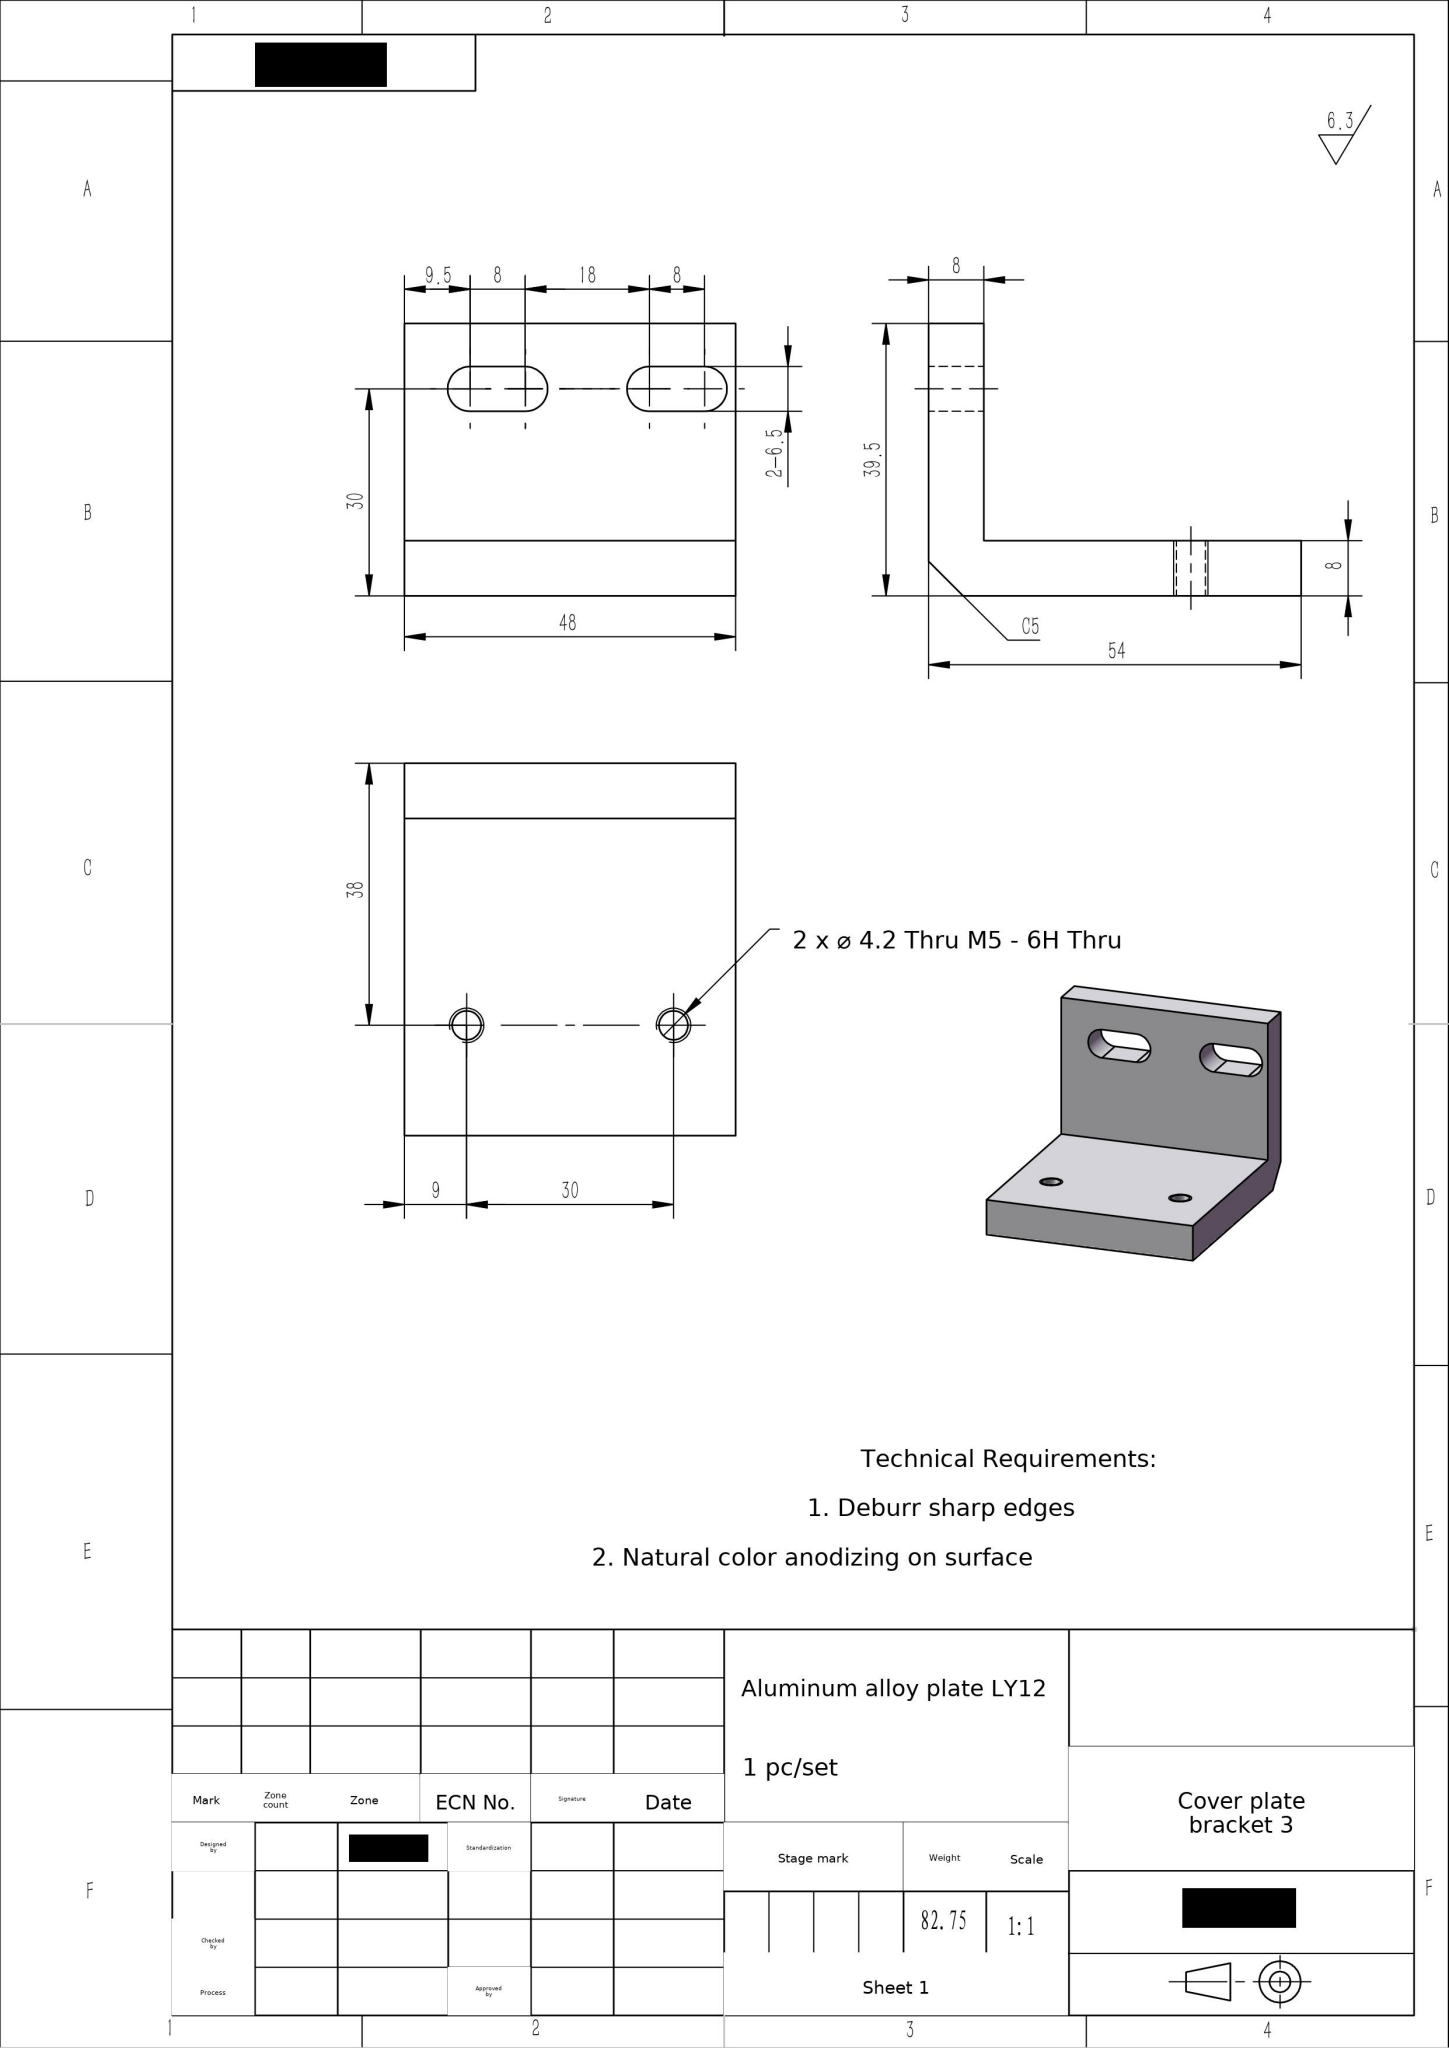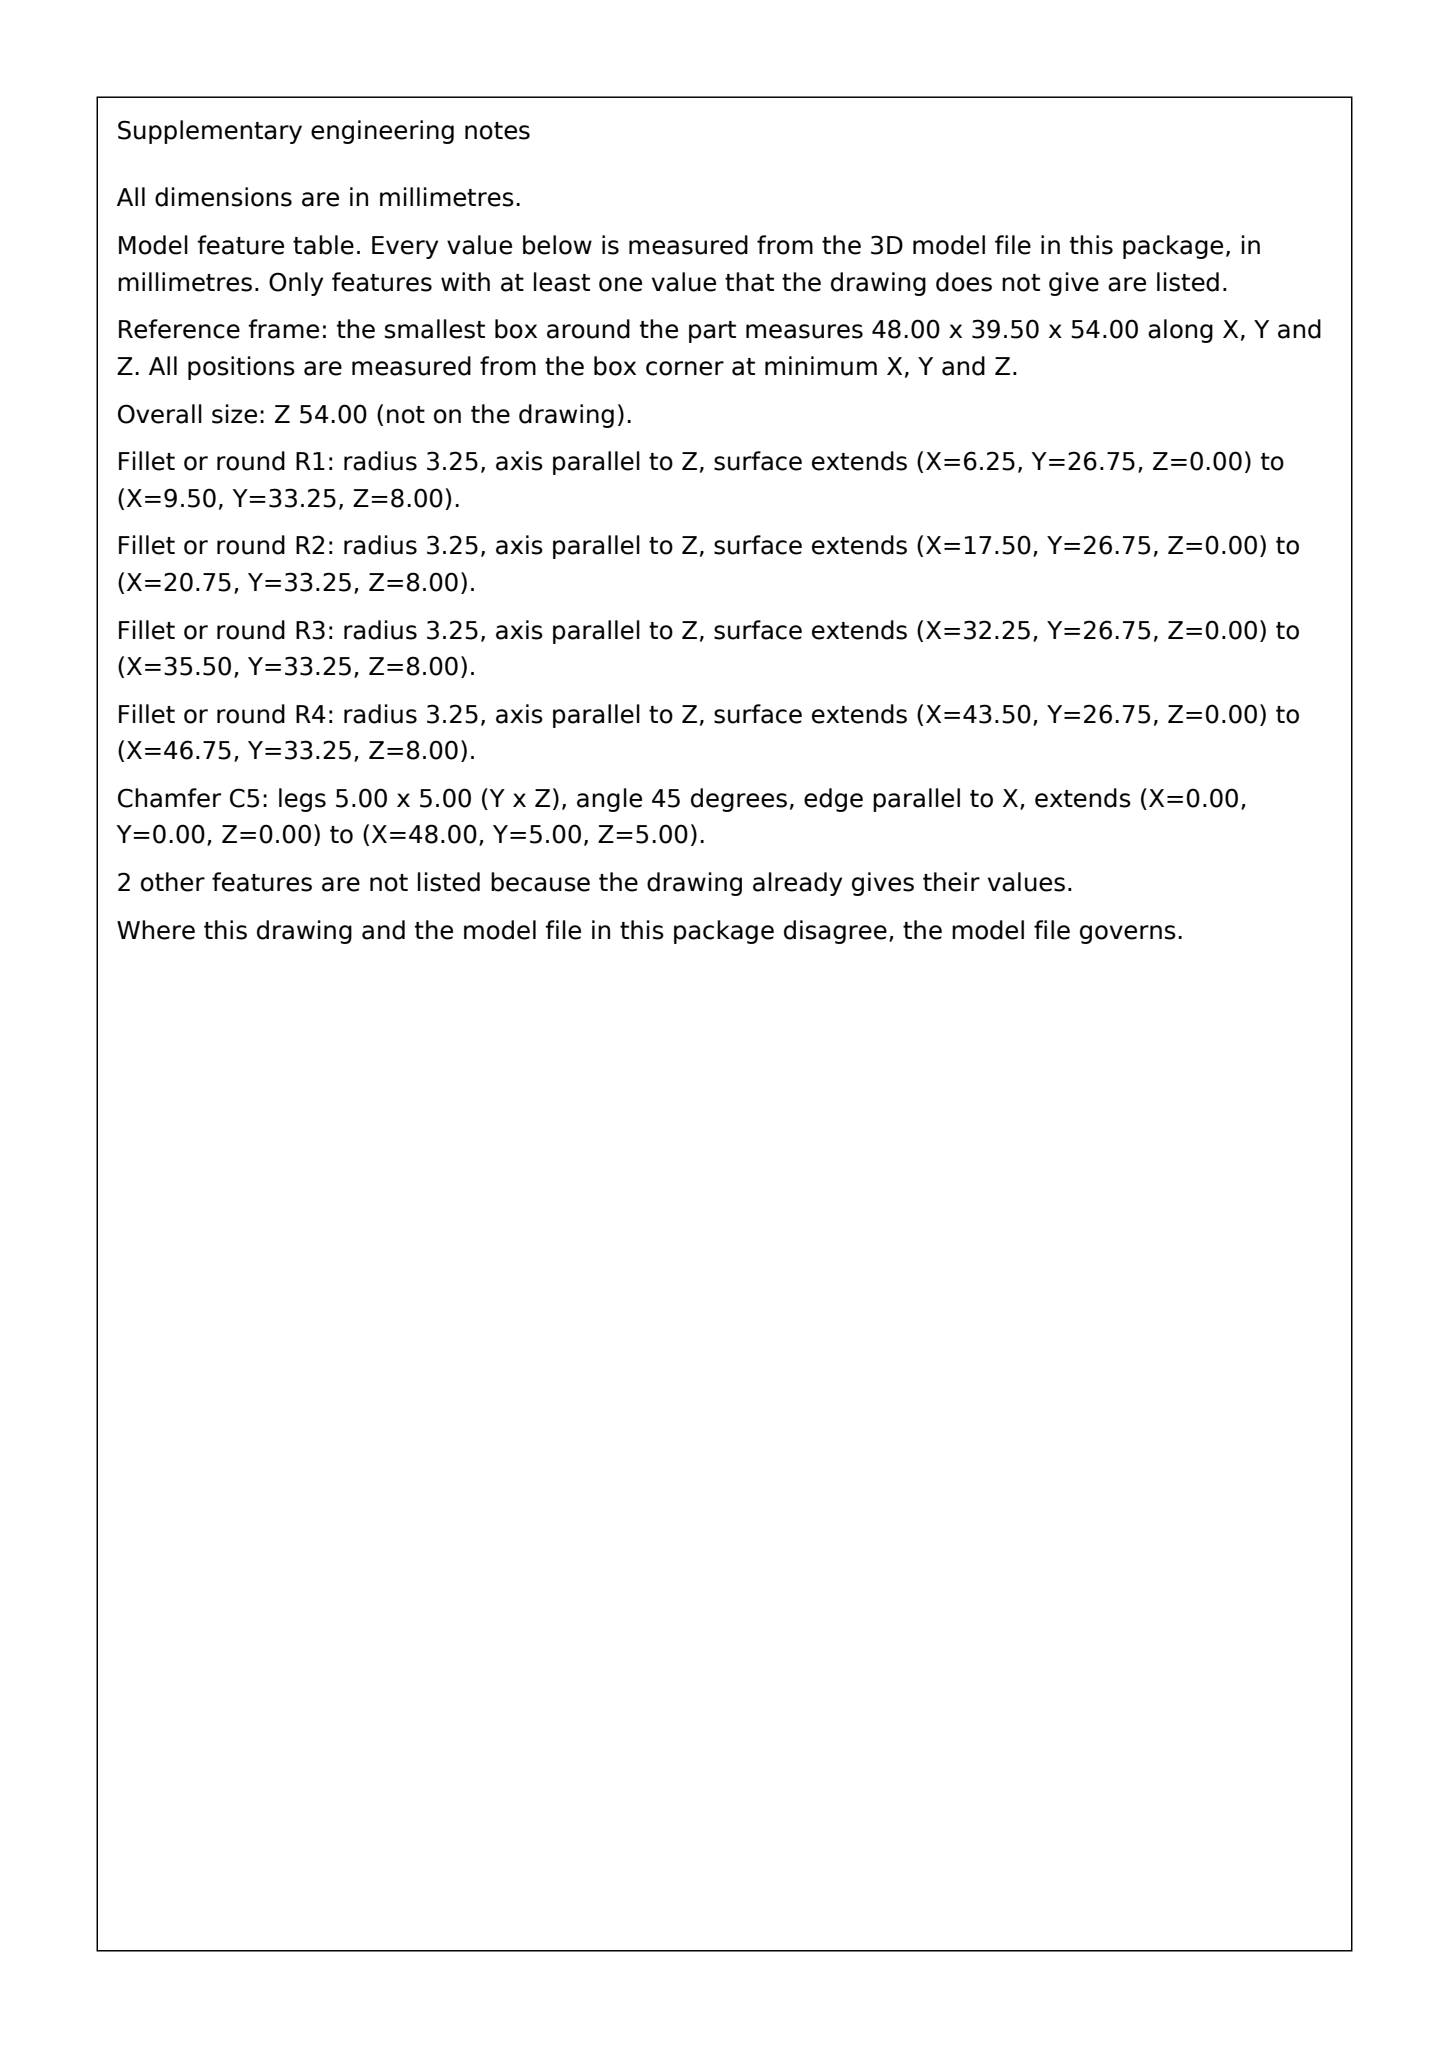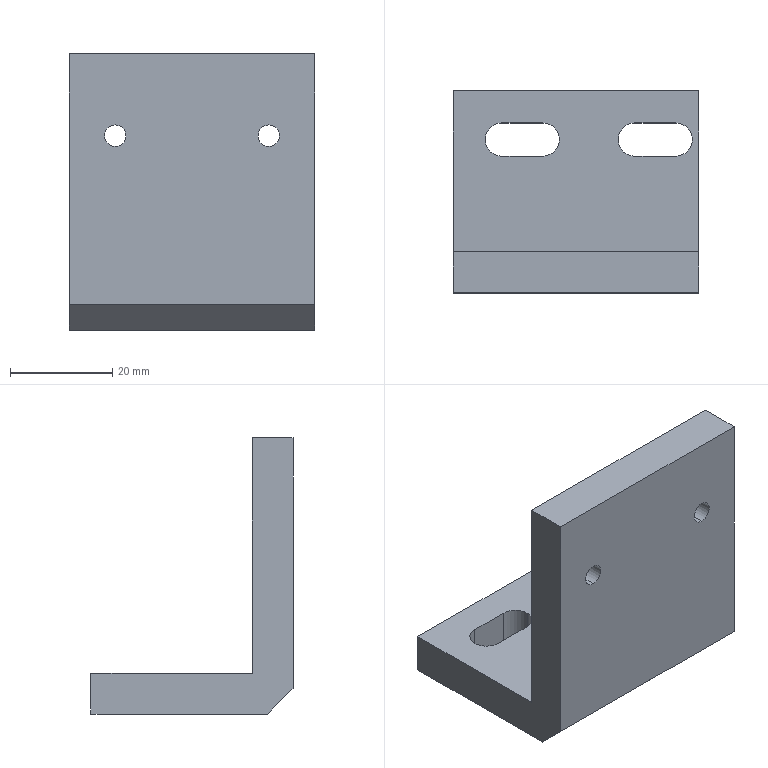Part | SolidWorks | mm | material Aluminum alloy plate LY12 | 1 solid | 23 faces | box 48 x 39.5 x 54 mm | volume 30647 mm3 | plane 13 | cylinder 10 | commonest cylinder face diameters 6.5 x6 4.2 x4
build123d program:
from build123d import *

# Parameters (mm, degrees)
BOSS_EXTRUDE1_DEPTH            = 27.5
CUT_EXTRUDE1_DEPTH             = 72.723
SKETCH4_W                      = 55
SKETCH4_H                      = 14
BOSS_EXTRUDE2_DEPTH            = 6
F_5_5_5_5_DIAMETER_HOLE2_D     = 5.5
F_5_5_5_5_DIAMETER_HOLE2_DEPTH = 6
SKETCH7_W                      = 7
SKETCH7_H                      = 30
CUT_EXTRUDE2_DEPTH             = 79.334
SKETCH8_W                      = 55
SKETCH8_H                      = 36
CUT_EXTRUDE3_DEPTH             = 79.334
MOVE_FACE1_BY                  = 8
MOVE_FACE1_2_BY                = 8
MOVE_FACE2_BY                  = 0.5
MOVE_FACE3_BY                  = 24
M5_TAPPED_HOLE1_D              = 4.2
CHAMFER1_SIZE                  = 5


with BuildPart() as part:
    # Sketch2 → Boss-Extrude1 (new, symmetric)
    with BuildSketch(Plane(origin=(0, 0, 0), x_dir=(0, 0, -1), z_dir=(1, 0, 0))):
        Polygon((0, 0), (0, 32), (-8, 32), (-8, 8), (-66, 8), (-66, 0), align=None)
    extrude(amount=BOSS_EXTRUDE1_DEPTH, both=True)

    # Sketch3 → Cut-Extrude1 (cut, through all)
    with BuildSketch(Plane.XY.offset(8)):
        with BuildLine():
            Line((8, 25.25), (16, 25.25))
            ThreePointArc((16, 25.25), (19.25, 22), (16, 18.75))
            Line((16, 18.75), (8, 18.75))
            ThreePointArc((8, 18.75), (4.75, 22), (8, 25.25))
        make_face()
        with BuildLine():
            Line((-18, 25.25), (-10, 25.25))
            ThreePointArc((-10, 25.25), (-6.75, 22), (-10, 18.75))
            Line((-10, 18.75), (-18, 18.75))
            ThreePointArc((-18, 18.75), (-21.25, 22), (-18, 25.25))
        make_face()
    extrude(amount=-CUT_EXTRUDE1_DEPTH, mode=Mode.SUBTRACT)

    # Sketch4 → Boss-Extrude2 (add)
    with BuildSketch(Plane.XY.offset(66)):
        with Locations((0, 15)):
            Rectangle(SKETCH4_W, SKETCH4_H)
    extrude(amount=-BOSS_EXTRUDE2_DEPTH)

    # 5.5 _5.5_ Diameter Hole2
    with Locations(Plane.XY.offset(66)):
        with Locations((-12.5, 15), (20, 15)):
            Hole(F_5_5_5_5_DIAMETER_HOLE2_D / 2, depth=F_5_5_5_5_DIAMETER_HOLE2_DEPTH)

    # Sketch7 → Cut-Extrude2 (cut, through all)
    with BuildSketch(Plane(origin=(0, 32, 0), x_dir=(1, 0, 0), z_dir=(0, 1, 0))):
        with Locations((24, -15)):
            Rectangle(SKETCH7_W, SKETCH7_H)
    extrude(amount=-CUT_EXTRUDE2_DEPTH, mode=Mode.SUBTRACT)

    # Sketch8 → Cut-Extrude3 (cut, through all)
    with BuildSketch(Plane(origin=(0, 32, 0), x_dir=(1, 0, 0), z_dir=(0, 1, 0))):
        with Locations((0, -48)):
            Rectangle(SKETCH8_W, SKETCH8_H)
    extrude(amount=-CUT_EXTRUDE3_DEPTH, mode=Mode.SUBTRACT)

    # Move Face1: a face moved outward by 8.0
    extrude(part.faces().sort_by_distance((-3.5, 0, 15))[0], amount=MOVE_FACE1_BY, dir=(0, -1, 0))

    # Move Face1 2: a face moved inward by 8.0
    extrude(part.faces().sort_by_distance((-3.5, 8, 19))[0], amount=MOVE_FACE1_2_BY, dir=(0, -1, 0), mode=Mode.SUBTRACT)

    # Move Face2: a face moved inward by 0.5
    extrude(part.faces().sort_by_distance((-3.5, 32, 4))[0], amount=MOVE_FACE2_BY, dir=(0, -1, 0), mode=Mode.SUBTRACT)

    # Move Face3: a face moved outward by 24.0
    extrude(part.faces().sort_by_distance((-3.5, -4, 30))[0], amount=MOVE_FACE3_BY, dir=(0, 0, 1))

    # M5 Tapped Hole1 (through all)
    with Locations(Plane(origin=(0, 0, 0), x_dir=(1, 0, 0), z_dir=(0, 1, 0))):
        with Locations((-18.5, -38), (11.5, -38)):
            Hole(M5_TAPPED_HOLE1_D / 2)

    # Chamfer1
    chamfer1_edges = [part.edges().sort_by_distance(p)[0] for p in [
        (-3.5, -8, 0),
    ]]
    chamfer(chamfer1_edges, length=CHAMFER1_SIZE)


solid = part.part
STEP:
#1=CARTESIAN_POINT('',(-18.5,-8.,35.9));
#2=VERTEX_POINT('',#1);
#3=CARTESIAN_POINT('',(-18.5,-8.,40.1));
#4=VERTEX_POINT('',#3);
#5=CARTESIAN_POINT('',(-18.5,-8.,38.));
#6=DIRECTION('',(0.,1.,0.));
#7=DIRECTION('',(0.,0.,1.));
#8=AXIS2_PLACEMENT_3D('',#5,#6,#7);
#9=CIRCLE('',#8,2.1);
#10=EDGE_CURVE('',#2,#4,#9,.T.);
#11=ORIENTED_EDGE('',*,*,#10,.F.);
#12=CARTESIAN_POINT('',(-18.5,-0.,35.9));
#13=VERTEX_POINT('',#12);
#14=CARTESIAN_POINT('',(-18.5,-0.,35.9));
#15=DIRECTION('',(0.,1.,0.));
#16=VECTOR('',#15,1000.);
#17=LINE('',#14,#16);
#18=EDGE_CURVE('',#2,#13,#17,.T.);
#19=ORIENTED_EDGE('',*,*,#18,.T.);
#20=CARTESIAN_POINT('',(-18.5,-0.,40.1));
#21=VERTEX_POINT('',#20);
#22=CARTESIAN_POINT('',(-18.5,-0.,38.));
#23=DIRECTION('',(0.,1.,0.));
#24=DIRECTION('',(0.,-0.,1.));
#25=AXIS2_PLACEMENT_3D('',#22,#23,#24);
#26=CIRCLE('',#25,2.1);
#27=EDGE_CURVE('',#13,#21,#26,.T.);
#28=ORIENTED_EDGE('',*,*,#27,.T.);
#29=CARTESIAN_POINT('',(-18.5,-0.,40.1));
#30=DIRECTION('',(0.,1.,0.));
#31=VECTOR('',#30,1000.);
#32=LINE('',#29,#31);
#33=EDGE_CURVE('',#4,#21,#32,.T.);
#34=ORIENTED_EDGE('',*,*,#33,.F.);
#35=EDGE_LOOP('',(#11,#19,#28,#34));
#36=FACE_OUTER_BOUND('',#35,.T.);
#37=CARTESIAN_POINT('',(-18.5,-0.,38.));
#38=DIRECTION('',(0.,1.,0.));
#39=DIRECTION('',(0.,-0.,1.));
#40=AXIS2_PLACEMENT_3D('',#37,#38,#39);
#41=CYLINDRICAL_SURFACE('',#40,2.1);
#42=ADVANCED_FACE('',(#36),#41,.F.);
#43=CARTESIAN_POINT('',(11.5,-8.,35.9));
#44=VERTEX_POINT('',#43);
#45=CARTESIAN_POINT('',(11.5,-8.,40.1));
#46=VERTEX_POINT('',#45);
#47=CARTESIAN_POINT('',(11.5,-8.,38.));
#48=DIRECTION('',(0.,1.,0.));
#49=DIRECTION('',(0.,0.,1.));
#50=AXIS2_PLACEMENT_3D('',#47,#48,#49);
#51=CIRCLE('',#50,2.1);
#52=EDGE_CURVE('',#44,#46,#51,.T.);
#53=ORIENTED_EDGE('',*,*,#52,.F.);
#54=CARTESIAN_POINT('',(11.5,-0.,35.9));
#55=VERTEX_POINT('',#54);
#56=CARTESIAN_POINT('',(11.5,-0.,35.9));
#57=DIRECTION('',(0.,1.,0.));
#58=VECTOR('',#57,1000.);
#59=LINE('',#56,#58);
#60=EDGE_CURVE('',#44,#55,#59,.T.);
#61=ORIENTED_EDGE('',*,*,#60,.T.);
#62=CARTESIAN_POINT('',(11.5,-0.,40.1));
#63=VERTEX_POINT('',#62);
#64=CARTESIAN_POINT('',(11.5,-0.,38.));
#65=DIRECTION('',(0.,1.,0.));
#66=DIRECTION('',(0.,-0.,1.));
#67=AXIS2_PLACEMENT_3D('',#64,#65,#66);
#68=CIRCLE('',#67,2.1);
#69=EDGE_CURVE('',#55,#63,#68,.T.);
#70=ORIENTED_EDGE('',*,*,#69,.T.);
#71=CARTESIAN_POINT('',(11.5,-0.,40.1));
#72=DIRECTION('',(0.,1.,0.));
#73=VECTOR('',#72,1000.);
#74=LINE('',#71,#73);
#75=EDGE_CURVE('',#46,#63,#74,.T.);
#76=ORIENTED_EDGE('',*,*,#75,.F.);
#77=EDGE_LOOP('',(#53,#61,#70,#76));
#78=FACE_OUTER_BOUND('',#77,.T.);
#79=CARTESIAN_POINT('',(11.5,-0.,38.));
#80=DIRECTION('',(0.,1.,0.));
#81=DIRECTION('',(0.,-0.,1.));
#82=AXIS2_PLACEMENT_3D('',#79,#80,#81);
#83=CYLINDRICAL_SURFACE('',#82,2.1);
#84=ADVANCED_FACE('',(#78),#83,.F.);
#85=CARTESIAN_POINT('',(19.25,22.,0.));
#86=VERTEX_POINT('',#85);
#87=CARTESIAN_POINT('',(16.,25.25,0.));
#88=VERTEX_POINT('',#87);
#89=CARTESIAN_POINT('',(16.,22.,0.));
#90=DIRECTION('',(0.,0.,1.));
#91=DIRECTION('',(1.,0.,0.));
#92=AXIS2_PLACEMENT_3D('',#89,#90,#91);
#93=CIRCLE('',#92,3.25);
#94=EDGE_CURVE('',#86,#88,#93,.T.);
#95=ORIENTED_EDGE('',*,*,#94,.F.);
#96=CARTESIAN_POINT('',(19.25,22.,8.));
#97=VERTEX_POINT('',#96);
#98=CARTESIAN_POINT('',(19.25,22.,0.));
#99=DIRECTION('',(0.,0.,1.));
#100=VECTOR('',#99,1000.);
#101=LINE('',#98,#100);
#102=EDGE_CURVE('',#86,#97,#101,.T.);
#103=ORIENTED_EDGE('',*,*,#102,.T.);
#104=CARTESIAN_POINT('',(16.,25.25,8.));
#105=VERTEX_POINT('',#104);
#106=CARTESIAN_POINT('',(16.,22.,8.));
#107=DIRECTION('',(0.,0.,1.));
#108=DIRECTION('',(1.,0.,0.));
#109=AXIS2_PLACEMENT_3D('',#106,#107,#108);
#110=CIRCLE('',#109,3.25);
#111=EDGE_CURVE('',#97,#105,#110,.T.);
#112=ORIENTED_EDGE('',*,*,#111,.T.);
#113=CARTESIAN_POINT('',(16.,25.25,0.));
#114=DIRECTION('',(0.,0.,1.));
#115=VECTOR('',#114,1000.);
#116=LINE('',#113,#115);
#117=EDGE_CURVE('',#88,#105,#116,.T.);
#118=ORIENTED_EDGE('',*,*,#117,.F.);
#119=EDGE_LOOP('',(#95,#103,#112,#118));
#120=FACE_OUTER_BOUND('',#119,.T.);
#121=CARTESIAN_POINT('',(16.,22.,0.));
#122=DIRECTION('',(0.,0.,1.));
#123=DIRECTION('',(1.,0.,0.));
#124=AXIS2_PLACEMENT_3D('',#121,#122,#123);
#125=CYLINDRICAL_SURFACE('',#124,3.25);
#126=ADVANCED_FACE('',(#120),#125,.F.);
#127=CARTESIAN_POINT('',(-6.75,22.,0.));
#128=VERTEX_POINT('',#127);
#129=CARTESIAN_POINT('',(-10.,25.25,0.));
#130=VERTEX_POINT('',#129);
#131=CARTESIAN_POINT('',(-10.,22.,0.));
#132=DIRECTION('',(0.,0.,1.));
#133=DIRECTION('',(1.,0.,0.));
#134=AXIS2_PLACEMENT_3D('',#131,#132,#133);
#135=CIRCLE('',#134,3.25);
#136=EDGE_CURVE('',#128,#130,#135,.T.);
#137=ORIENTED_EDGE('',*,*,#136,.F.);
#138=CARTESIAN_POINT('',(-6.75,22.,8.));
#139=VERTEX_POINT('',#138);
#140=CARTESIAN_POINT('',(-6.75,22.,0.));
#141=DIRECTION('',(0.,0.,1.));
#142=VECTOR('',#141,1000.);
#143=LINE('',#140,#142);
#144=EDGE_CURVE('',#128,#139,#143,.T.);
#145=ORIENTED_EDGE('',*,*,#144,.T.);
#146=CARTESIAN_POINT('',(-10.,25.25,8.));
#147=VERTEX_POINT('',#146);
#148=CARTESIAN_POINT('',(-10.,22.,8.));
#149=DIRECTION('',(0.,0.,1.));
#150=DIRECTION('',(1.,0.,0.));
#151=AXIS2_PLACEMENT_3D('',#148,#149,#150);
#152=CIRCLE('',#151,3.25);
#153=EDGE_CURVE('',#139,#147,#152,.T.);
#154=ORIENTED_EDGE('',*,*,#153,.T.);
#155=CARTESIAN_POINT('',(-10.,25.25,0.));
#156=DIRECTION('',(0.,0.,1.));
#157=VECTOR('',#156,1000.);
#158=LINE('',#155,#157);
#159=EDGE_CURVE('',#130,#147,#158,.T.);
#160=ORIENTED_EDGE('',*,*,#159,.F.);
#161=EDGE_LOOP('',(#137,#145,#154,#160));
#162=FACE_OUTER_BOUND('',#161,.T.);
#163=CARTESIAN_POINT('',(-10.,22.,0.));
#164=DIRECTION('',(0.,0.,1.));
#165=DIRECTION('',(1.,0.,0.));
#166=AXIS2_PLACEMENT_3D('',#163,#164,#165);
#167=CYLINDRICAL_SURFACE('',#166,3.25);
#168=ADVANCED_FACE('',(#162),#167,.F.);
#169=CARTESIAN_POINT('',(-18.5,-8.,38.));
#170=DIRECTION('',(0.,1.,0.));
#171=DIRECTION('',(0.,0.,1.));
#172=AXIS2_PLACEMENT_3D('',#169,#170,#171);
#173=CIRCLE('',#172,2.1);
#174=EDGE_CURVE('',#4,#2,#173,.T.);
#175=ORIENTED_EDGE('',*,*,#174,.T.);
#176=ORIENTED_EDGE('',*,*,#10,.T.);
#177=EDGE_LOOP('',(#175,#176));
#178=FACE_BOUND('',#177,.T.);
#179=CARTESIAN_POINT('',(11.5,-8.,38.));
#180=DIRECTION('',(0.,1.,0.));
#181=DIRECTION('',(0.,0.,1.));
#182=AXIS2_PLACEMENT_3D('',#179,#180,#181);
#183=CIRCLE('',#182,2.1);
#184=EDGE_CURVE('',#46,#44,#183,.T.);
#185=ORIENTED_EDGE('',*,*,#184,.T.);
#186=ORIENTED_EDGE('',*,*,#52,.T.);
#187=EDGE_LOOP('',(#185,#186));
#188=FACE_BOUND('',#187,.T.);
#189=CARTESIAN_POINT('',(-27.5,-8.,54.));
#190=VERTEX_POINT('',#189);
#191=CARTESIAN_POINT('',(-27.5,-8.,5.));
#192=VERTEX_POINT('',#191);
#193=CARTESIAN_POINT('',(-27.5,-8.,66.));
#194=DIRECTION('',(0.,0.,-1.));
#195=VECTOR('',#194,1000.);
#196=LINE('',#193,#195);
#197=EDGE_CURVE('',#190,#192,#196,.T.);
#198=ORIENTED_EDGE('',*,*,#197,.T.);
#199=CARTESIAN_POINT('',(20.5,-8.,5.));
#200=VERTEX_POINT('',#199);
#201=CARTESIAN_POINT('',(27.5,-8.,5.));
#202=DIRECTION('',(1.,0.,0.));
#203=VECTOR('',#202,1000.);
#204=LINE('',#201,#203);
#205=EDGE_CURVE('',#192,#200,#204,.T.);
#206=ORIENTED_EDGE('',*,*,#205,.T.);
#207=CARTESIAN_POINT('',(20.5,-8.,54.));
#208=VERTEX_POINT('',#207);
#209=CARTESIAN_POINT('',(20.5,-8.,0.));
#210=DIRECTION('',(0.,0.,1.));
#211=VECTOR('',#210,1000.);
#212=LINE('',#209,#211);
#213=EDGE_CURVE('',#200,#208,#212,.T.);
#214=ORIENTED_EDGE('',*,*,#213,.T.);
#215=CARTESIAN_POINT('',(27.5,-8.,54.));
#216=DIRECTION('',(-1.,0.,0.));
#217=VECTOR('',#216,1000.);
#218=LINE('',#215,#217);
#219=EDGE_CURVE('',#208,#190,#218,.T.);
#220=ORIENTED_EDGE('',*,*,#219,.T.);
#221=EDGE_LOOP('',(#198,#206,#214,#220));
#222=FACE_OUTER_BOUND('',#221,.T.);
#223=CARTESIAN_POINT('',(27.5,-8.,66.));
#224=DIRECTION('',(0.,1.,0.));
#225=DIRECTION('',(0.,0.,1.));
#226=AXIS2_PLACEMENT_3D('',#223,#224,#225);
#227=PLANE('',#226);
#228=ADVANCED_FACE('',(#178,#188,#222),#227,.F.);
#229=CARTESIAN_POINT('',(8.,25.25,0.));
#230=VERTEX_POINT('',#229);
#231=CARTESIAN_POINT('',(8.,25.25,0.));
#232=DIRECTION('',(-1.,-0.,0.));
#233=VECTOR('',#232,1000.);
#234=LINE('',#231,#233);
#235=EDGE_CURVE('',#88,#230,#234,.T.);
#236=ORIENTED_EDGE('',*,*,#235,.T.);
#237=CARTESIAN_POINT('',(8.,18.75,0.));
#238=VERTEX_POINT('',#237);
#239=CARTESIAN_POINT('',(8.,22.,0.));
#240=DIRECTION('',(0.,0.,1.));
#241=DIRECTION('',(1.,0.,0.));
#242=AXIS2_PLACEMENT_3D('',#239,#240,#241);
#243=CIRCLE('',#242,3.25);
#244=EDGE_CURVE('',#230,#238,#243,.T.);
#245=ORIENTED_EDGE('',*,*,#244,.T.);
#246=CARTESIAN_POINT('',(16.,18.75,0.));
#247=VERTEX_POINT('',#246);
#248=CARTESIAN_POINT('',(8.,18.75,0.));
#249=DIRECTION('',(1.,0.,0.));
#250=VECTOR('',#249,1000.);
#251=LINE('',#248,#250);
#252=EDGE_CURVE('',#238,#247,#251,.T.);
#253=ORIENTED_EDGE('',*,*,#252,.T.);
#254=CARTESIAN_POINT('',(16.,22.,0.));
#255=DIRECTION('',(0.,0.,1.));
#256=DIRECTION('',(1.,0.,0.));
#257=AXIS2_PLACEMENT_3D('',#254,#255,#256);
#258=CIRCLE('',#257,3.25);
#259=EDGE_CURVE('',#247,#86,#258,.T.);
#260=ORIENTED_EDGE('',*,*,#259,.T.);
#261=ORIENTED_EDGE('',*,*,#94,.T.);
#262=EDGE_LOOP('',(#236,#245,#253,#260,#261));
#263=FACE_BOUND('',#262,.T.);
#264=CARTESIAN_POINT('',(-18.,25.25,0.));
#265=VERTEX_POINT('',#264);
#266=CARTESIAN_POINT('',(-18.,25.25,0.));
#267=DIRECTION('',(-1.,0.,0.));
#268=VECTOR('',#267,1000.);
#269=LINE('',#266,#268);
#270=EDGE_CURVE('',#130,#265,#269,.T.);
#271=ORIENTED_EDGE('',*,*,#270,.T.);
#272=CARTESIAN_POINT('',(-18.,18.75,0.));
#273=VERTEX_POINT('',#272);
#274=CARTESIAN_POINT('',(-18.,22.,0.));
#275=DIRECTION('',(0.,0.,1.));
#276=DIRECTION('',(1.,0.,0.));
#277=AXIS2_PLACEMENT_3D('',#274,#275,#276);
#278=CIRCLE('',#277,3.25);
#279=EDGE_CURVE('',#265,#273,#278,.T.);
#280=ORIENTED_EDGE('',*,*,#279,.T.);
#281=CARTESIAN_POINT('',(-10.,18.75,0.));
#282=VERTEX_POINT('',#281);
#283=CARTESIAN_POINT('',(-18.,18.75,0.));
#284=DIRECTION('',(1.,0.,0.));
#285=VECTOR('',#284,1000.);
#286=LINE('',#283,#285);
#287=EDGE_CURVE('',#273,#282,#286,.T.);
#288=ORIENTED_EDGE('',*,*,#287,.T.);
#289=CARTESIAN_POINT('',(-10.,22.,0.));
#290=DIRECTION('',(0.,0.,1.));
#291=DIRECTION('',(1.,0.,0.));
#292=AXIS2_PLACEMENT_3D('',#289,#290,#291);
#293=CIRCLE('',#292,3.25);
#294=EDGE_CURVE('',#282,#128,#293,.T.);
#295=ORIENTED_EDGE('',*,*,#294,.T.);
#296=ORIENTED_EDGE('',*,*,#136,.T.);
#297=EDGE_LOOP('',(#271,#280,#288,#295,#296));
#298=FACE_BOUND('',#297,.T.);
#299=CARTESIAN_POINT('',(20.5,-3.,0.));
#300=VERTEX_POINT('',#299);
#301=CARTESIAN_POINT('',(20.5,31.5,0.));
#302=VERTEX_POINT('',#301);
#303=CARTESIAN_POINT('',(20.5,0.,0.));
#304=DIRECTION('',(0.,1.,0.));
#305=VECTOR('',#304,1000.);
#306=LINE('',#303,#305);
#307=EDGE_CURVE('',#300,#302,#306,.T.);
#308=ORIENTED_EDGE('',*,*,#307,.F.);
#309=CARTESIAN_POINT('',(-27.5,-3.,0.));
#310=VERTEX_POINT('',#309);
#311=CARTESIAN_POINT('',(27.5,-3.,0.));
#312=DIRECTION('',(-1.,0.,0.));
#313=VECTOR('',#312,1000.);
#314=LINE('',#311,#313);
#315=EDGE_CURVE('',#300,#310,#314,.T.);
#316=ORIENTED_EDGE('',*,*,#315,.T.);
#317=CARTESIAN_POINT('',(-27.5,31.5,0.));
#318=VERTEX_POINT('',#317);
#319=CARTESIAN_POINT('',(-27.5,0.,0.));
#320=DIRECTION('',(0.,1.,0.));
#321=VECTOR('',#320,1000.);
#322=LINE('',#319,#321);
#323=EDGE_CURVE('',#310,#318,#322,.T.);
#324=ORIENTED_EDGE('',*,*,#323,.T.);
#325=CARTESIAN_POINT('',(27.5,31.5,0.));
#326=DIRECTION('',(-1.,0.,0.));
#327=VECTOR('',#326,1000.);
#328=LINE('',#325,#327);
#329=EDGE_CURVE('',#302,#318,#328,.T.);
#330=ORIENTED_EDGE('',*,*,#329,.F.);
#331=EDGE_LOOP('',(#308,#316,#324,#330));
#332=FACE_OUTER_BOUND('',#331,.T.);
#333=CARTESIAN_POINT('',(27.5,0.,0.));
#334=DIRECTION('',(0.,0.,1.));
#335=DIRECTION('',(1.,0.,0.));
#336=AXIS2_PLACEMENT_3D('',#333,#334,#335);
#337=PLANE('',#336);
#338=ADVANCED_FACE('',(#263,#298,#332),#337,.F.);
#339=CARTESIAN_POINT('',(20.5,31.5,8.));
#340=VERTEX_POINT('',#339);
#341=CARTESIAN_POINT('',(-27.5,31.5,8.));
#342=VERTEX_POINT('',#341);
#343=CARTESIAN_POINT('',(27.5,31.5,8.));
#344=DIRECTION('',(-1.,0.,0.));
#345=VECTOR('',#344,1000.);
#346=LINE('',#343,#345);
#347=EDGE_CURVE('',#340,#342,#346,.T.);
#348=ORIENTED_EDGE('',*,*,#347,.F.);
#349=CARTESIAN_POINT('',(20.5,31.5,0.));
#350=DIRECTION('',(0.,0.,1.));
#351=VECTOR('',#350,1000.);
#352=LINE('',#349,#351);
#353=EDGE_CURVE('',#302,#340,#352,.T.);
#354=ORIENTED_EDGE('',*,*,#353,.F.);
#355=ORIENTED_EDGE('',*,*,#329,.T.);
#356=CARTESIAN_POINT('',(-27.5,31.5,0.));
#357=DIRECTION('',(0.,0.,1.));
#358=VECTOR('',#357,1000.);
#359=LINE('',#356,#358);
#360=EDGE_CURVE('',#318,#342,#359,.T.);
#361=ORIENTED_EDGE('',*,*,#360,.T.);
#362=EDGE_LOOP('',(#348,#354,#355,#361));
#363=FACE_OUTER_BOUND('',#362,.T.);
#364=CARTESIAN_POINT('',(27.5,31.5,0.));
#365=DIRECTION('',(0.,-1.,0.));
#366=DIRECTION('',(0.,0.,-1.));
#367=AXIS2_PLACEMENT_3D('',#364,#365,#366);
#368=PLANE('',#367);
#369=ADVANCED_FACE('',(#363),#368,.F.);
#370=CARTESIAN_POINT('',(8.,18.75,8.));
#371=VERTEX_POINT('',#370);
#372=CARTESIAN_POINT('',(16.,18.75,8.));
#373=VERTEX_POINT('',#372);
#374=CARTESIAN_POINT('',(8.,18.75,8.));
#375=DIRECTION('',(1.,0.,0.));
#376=VECTOR('',#375,1000.);
#377=LINE('',#374,#376);
#378=EDGE_CURVE('',#371,#373,#377,.T.);
#379=ORIENTED_EDGE('',*,*,#378,.F.);
#380=CARTESIAN_POINT('',(8.,25.25,8.));
#381=VERTEX_POINT('',#380);
#382=CARTESIAN_POINT('',(8.,22.,8.));
#383=DIRECTION('',(0.,0.,1.));
#384=DIRECTION('',(1.,0.,0.));
#385=AXIS2_PLACEMENT_3D('',#382,#383,#384);
#386=CIRCLE('',#385,3.25);
#387=EDGE_CURVE('',#381,#371,#386,.T.);
#388=ORIENTED_EDGE('',*,*,#387,.F.);
#389=CARTESIAN_POINT('',(8.,25.25,8.));
#390=DIRECTION('',(-1.,-0.,0.));
#391=VECTOR('',#390,1000.);
#392=LINE('',#389,#391);
#393=EDGE_CURVE('',#105,#381,#392,.T.);
#394=ORIENTED_EDGE('',*,*,#393,.F.);
#395=ORIENTED_EDGE('',*,*,#111,.F.);
#396=CARTESIAN_POINT('',(16.,22.,8.));
#397=DIRECTION('',(0.,0.,1.));
#398=DIRECTION('',(1.,0.,0.));
#399=AXIS2_PLACEMENT_3D('',#396,#397,#398);
#400=CIRCLE('',#399,3.25);
#401=EDGE_CURVE('',#373,#97,#400,.T.);
#402=ORIENTED_EDGE('',*,*,#401,.F.);
#403=EDGE_LOOP('',(#379,#388,#394,#395,#402));
#404=FACE_BOUND('',#403,.T.);
#405=CARTESIAN_POINT('',(-18.,18.75,8.));
#406=VERTEX_POINT('',#405);
#407=CARTESIAN_POINT('',(-10.,18.75,8.));
#408=VERTEX_POINT('',#407);
#409=CARTESIAN_POINT('',(-18.,18.75,8.));
#410=DIRECTION('',(1.,0.,0.));
#411=VECTOR('',#410,1000.);
#412=LINE('',#409,#411);
#413=EDGE_CURVE('',#406,#408,#412,.T.);
#414=ORIENTED_EDGE('',*,*,#413,.F.);
#415=CARTESIAN_POINT('',(-18.,25.25,8.));
#416=VERTEX_POINT('',#415);
#417=CARTESIAN_POINT('',(-18.,22.,8.));
#418=DIRECTION('',(0.,0.,1.));
#419=DIRECTION('',(1.,0.,0.));
#420=AXIS2_PLACEMENT_3D('',#417,#418,#419);
#421=CIRCLE('',#420,3.25);
#422=EDGE_CURVE('',#416,#406,#421,.T.);
#423=ORIENTED_EDGE('',*,*,#422,.F.);
#424=CARTESIAN_POINT('',(-18.,25.25,8.));
#425=DIRECTION('',(-1.,0.,0.));
#426=VECTOR('',#425,1000.);
#427=LINE('',#424,#426);
#428=EDGE_CURVE('',#147,#416,#427,.T.);
#429=ORIENTED_EDGE('',*,*,#428,.F.);
#430=ORIENTED_EDGE('',*,*,#153,.F.);
#431=CARTESIAN_POINT('',(-10.,22.,8.));
#432=DIRECTION('',(0.,0.,1.));
#433=DIRECTION('',(1.,0.,0.));
#434=AXIS2_PLACEMENT_3D('',#431,#432,#433);
#435=CIRCLE('',#434,3.25);
#436=EDGE_CURVE('',#408,#139,#435,.T.);
#437=ORIENTED_EDGE('',*,*,#436,.F.);
#438=EDGE_LOOP('',(#414,#423,#429,#430,#437));
#439=FACE_BOUND('',#438,.T.);
#440=CARTESIAN_POINT('',(20.5,0.,8.));
#441=VERTEX_POINT('',#440);
#442=CARTESIAN_POINT('',(-27.5,0.,8.));
#443=VERTEX_POINT('',#442);
#444=CARTESIAN_POINT('',(27.5,0.,8.));
#445=DIRECTION('',(-1.,0.,0.));
#446=VECTOR('',#445,1000.);
#447=LINE('',#444,#446);
#448=EDGE_CURVE('',#441,#443,#447,.T.);
#449=ORIENTED_EDGE('',*,*,#448,.F.);
#450=CARTESIAN_POINT('',(20.5,32.,8.));
#451=DIRECTION('',(0.,1.,0.));
#452=VECTOR('',#451,1000.);
#453=LINE('',#450,#452);
#454=EDGE_CURVE('',#441,#340,#453,.T.);
#455=ORIENTED_EDGE('',*,*,#454,.T.);
#456=ORIENTED_EDGE('',*,*,#347,.T.);
#457=CARTESIAN_POINT('',(-27.5,32.,8.));
#458=DIRECTION('',(0.,-1.,-0.));
#459=VECTOR('',#458,1000.);
#460=LINE('',#457,#459);
#461=EDGE_CURVE('',#342,#443,#460,.T.);
#462=ORIENTED_EDGE('',*,*,#461,.T.);
#463=EDGE_LOOP('',(#449,#455,#456,#462));
#464=FACE_OUTER_BOUND('',#463,.T.);
#465=CARTESIAN_POINT('',(27.5,32.,8.));
#466=DIRECTION('',(0.,0.,-1.));
#467=DIRECTION('',(0.,1.,0.));
#468=AXIS2_PLACEMENT_3D('',#465,#466,#467);
#469=PLANE('',#468);
#470=ADVANCED_FACE('',(#404,#439,#464),#469,.F.);
#471=CARTESIAN_POINT('',(-18.5,-0.,38.));
#472=DIRECTION('',(0.,1.,0.));
#473=DIRECTION('',(0.,-0.,1.));
#474=AXIS2_PLACEMENT_3D('',#471,#472,#473);
#475=CIRCLE('',#474,2.1);
#476=EDGE_CURVE('',#21,#13,#475,.T.);
#477=ORIENTED_EDGE('',*,*,#476,.F.);
#478=ORIENTED_EDGE('',*,*,#27,.F.);
#479=EDGE_LOOP('',(#477,#478));
#480=FACE_BOUND('',#479,.T.);
#481=CARTESIAN_POINT('',(11.5,-0.,38.));
#482=DIRECTION('',(0.,1.,0.));
#483=DIRECTION('',(0.,-0.,1.));
#484=AXIS2_PLACEMENT_3D('',#481,#482,#483);
#485=CIRCLE('',#484,2.1);
#486=EDGE_CURVE('',#63,#55,#485,.T.);
#487=ORIENTED_EDGE('',*,*,#486,.F.);
#488=ORIENTED_EDGE('',*,*,#69,.F.);
#489=EDGE_LOOP('',(#487,#488));
#490=FACE_BOUND('',#489,.T.);
#491=CARTESIAN_POINT('',(-27.5,0.,54.));
#492=VERTEX_POINT('',#491);
#493=CARTESIAN_POINT('',(-27.5,0.,8.));
#494=DIRECTION('',(0.,-0.,1.));
#495=VECTOR('',#494,1000.);
#496=LINE('',#493,#495);
#497=EDGE_CURVE('',#443,#492,#496,.T.);
#498=ORIENTED_EDGE('',*,*,#497,.T.);
#499=CARTESIAN_POINT('',(20.5,0.,54.));
#500=VERTEX_POINT('',#499);
#501=CARTESIAN_POINT('',(27.5,0.,54.));
#502=DIRECTION('',(1.,0.,0.));
#503=VECTOR('',#502,1000.);
#504=LINE('',#501,#503);
#505=EDGE_CURVE('',#492,#500,#504,.T.);
#506=ORIENTED_EDGE('',*,*,#505,.T.);
#507=CARTESIAN_POINT('',(20.5,0.,8.));
#508=DIRECTION('',(-0.,0.,-1.));
#509=VECTOR('',#508,1000.);
#510=LINE('',#507,#509);
#511=EDGE_CURVE('',#500,#441,#510,.T.);
#512=ORIENTED_EDGE('',*,*,#511,.T.);
#513=ORIENTED_EDGE('',*,*,#448,.T.);
#514=EDGE_LOOP('',(#498,#506,#512,#513));
#515=FACE_OUTER_BOUND('',#514,.T.);
#516=CARTESIAN_POINT('',(27.5,0.,8.));
#517=DIRECTION('',(0.,-1.,-0.));
#518=DIRECTION('',(0.,0.,-1.));
#519=AXIS2_PLACEMENT_3D('',#516,#517,#518);
#520=PLANE('',#519);
#521=ADVANCED_FACE('',(#480,#490,#515),#520,.F.);
#522=ORIENTED_EDGE('',*,*,#323,.F.);
#523=CARTESIAN_POINT('',(-27.5,-3.,0.));
#524=DIRECTION('',(0.,-0.7071,0.7071));
#525=VECTOR('',#524,1000.);
#526=LINE('',#523,#525);
#527=EDGE_CURVE('',#310,#192,#526,.T.);
#528=ORIENTED_EDGE('',*,*,#527,.T.);
#529=ORIENTED_EDGE('',*,*,#197,.F.);
#530=CARTESIAN_POINT('',(-27.5,0.,54.));
#531=DIRECTION('',(0.,1.,0.));
#532=VECTOR('',#531,1000.);
#533=LINE('',#530,#532);
#534=EDGE_CURVE('',#190,#492,#533,.T.);
#535=ORIENTED_EDGE('',*,*,#534,.T.);
#536=ORIENTED_EDGE('',*,*,#497,.F.);
#537=ORIENTED_EDGE('',*,*,#461,.F.);
#538=ORIENTED_EDGE('',*,*,#360,.F.);
#539=EDGE_LOOP('',(#522,#528,#529,#535,#536,#537,#538));
#540=FACE_OUTER_BOUND('',#539,.T.);
#541=CARTESIAN_POINT('',(-27.5,0.,0.));
#542=DIRECTION('',(1.,0.,0.));
#543=DIRECTION('',(0.,0.,-1.));
#544=AXIS2_PLACEMENT_3D('',#541,#542,#543);
#545=PLANE('',#544);
#546=ADVANCED_FACE('',(#540),#545,.F.);
#547=ORIENTED_EDGE('',*,*,#422,.T.);
#548=CARTESIAN_POINT('',(-18.,18.75,0.));
#549=DIRECTION('',(0.,0.,1.));
#550=VECTOR('',#549,1000.);
#551=LINE('',#548,#550);
#552=EDGE_CURVE('',#273,#406,#551,.T.);
#553=ORIENTED_EDGE('',*,*,#552,.F.);
#554=ORIENTED_EDGE('',*,*,#279,.F.);
#555=CARTESIAN_POINT('',(-18.,25.25,0.));
#556=DIRECTION('',(0.,0.,1.));
#557=VECTOR('',#556,1000.);
#558=LINE('',#555,#557);
#559=EDGE_CURVE('',#265,#416,#558,.T.);
#560=ORIENTED_EDGE('',*,*,#559,.T.);
#561=EDGE_LOOP('',(#547,#553,#554,#560));
#562=FACE_OUTER_BOUND('',#561,.T.);
#563=CARTESIAN_POINT('',(-18.,22.,0.));
#564=DIRECTION('',(0.,0.,1.));
#565=DIRECTION('',(1.,0.,0.));
#566=AXIS2_PLACEMENT_3D('',#563,#564,#565);
#567=CYLINDRICAL_SURFACE('',#566,3.25);
#568=ADVANCED_FACE('',(#562),#567,.F.);
#569=ORIENTED_EDGE('',*,*,#428,.T.);
#570=ORIENTED_EDGE('',*,*,#559,.F.);
#571=ORIENTED_EDGE('',*,*,#270,.F.);
#572=ORIENTED_EDGE('',*,*,#159,.T.);
#573=EDGE_LOOP('',(#569,#570,#571,#572));
#574=FACE_OUTER_BOUND('',#573,.T.);
#575=CARTESIAN_POINT('',(-18.,25.25,0.));
#576=DIRECTION('',(0.,1.,0.));
#577=DIRECTION('',(0.,0.,1.));
#578=AXIS2_PLACEMENT_3D('',#575,#576,#577);
#579=PLANE('',#578);
#580=ADVANCED_FACE('',(#574),#579,.F.);
#581=ORIENTED_EDGE('',*,*,#144,.F.);
#582=ORIENTED_EDGE('',*,*,#294,.F.);
#583=CARTESIAN_POINT('',(-10.,18.75,0.));
#584=DIRECTION('',(0.,0.,1.));
#585=VECTOR('',#584,1000.);
#586=LINE('',#583,#585);
#587=EDGE_CURVE('',#282,#408,#586,.T.);
#588=ORIENTED_EDGE('',*,*,#587,.T.);
#589=ORIENTED_EDGE('',*,*,#436,.T.);
#590=EDGE_LOOP('',(#581,#582,#588,#589));
#591=FACE_OUTER_BOUND('',#590,.T.);
#592=CARTESIAN_POINT('',(-10.,22.,0.));
#593=DIRECTION('',(0.,0.,1.));
#594=DIRECTION('',(1.,0.,0.));
#595=AXIS2_PLACEMENT_3D('',#592,#593,#594);
#596=CYLINDRICAL_SURFACE('',#595,3.25);
#597=ADVANCED_FACE('',(#591),#596,.F.);
#598=ORIENTED_EDGE('',*,*,#413,.T.);
#599=ORIENTED_EDGE('',*,*,#587,.F.);
#600=ORIENTED_EDGE('',*,*,#287,.F.);
#601=ORIENTED_EDGE('',*,*,#552,.T.);
#602=EDGE_LOOP('',(#598,#599,#600,#601));
#603=FACE_OUTER_BOUND('',#602,.T.);
#604=CARTESIAN_POINT('',(-18.,18.75,0.));
#605=DIRECTION('',(0.,-1.,0.));
#606=DIRECTION('',(0.,0.,-1.));
#607=AXIS2_PLACEMENT_3D('',#604,#605,#606);
#608=PLANE('',#607);
#609=ADVANCED_FACE('',(#603),#608,.F.);
#610=ORIENTED_EDGE('',*,*,#387,.T.);
#611=CARTESIAN_POINT('',(8.,18.75,0.));
#612=DIRECTION('',(0.,0.,1.));
#613=VECTOR('',#612,1000.);
#614=LINE('',#611,#613);
#615=EDGE_CURVE('',#238,#371,#614,.T.);
#616=ORIENTED_EDGE('',*,*,#615,.F.);
#617=ORIENTED_EDGE('',*,*,#244,.F.);
#618=CARTESIAN_POINT('',(8.,25.25,0.));
#619=DIRECTION('',(0.,0.,1.));
#620=VECTOR('',#619,1000.);
#621=LINE('',#618,#620);
#622=EDGE_CURVE('',#230,#381,#621,.T.);
#623=ORIENTED_EDGE('',*,*,#622,.T.);
#624=EDGE_LOOP('',(#610,#616,#617,#623));
#625=FACE_OUTER_BOUND('',#624,.T.);
#626=CARTESIAN_POINT('',(8.,22.,0.));
#627=DIRECTION('',(0.,0.,1.));
#628=DIRECTION('',(1.,0.,0.));
#629=AXIS2_PLACEMENT_3D('',#626,#627,#628);
#630=CYLINDRICAL_SURFACE('',#629,3.25);
#631=ADVANCED_FACE('',(#625),#630,.F.);
#632=ORIENTED_EDGE('',*,*,#393,.T.);
#633=ORIENTED_EDGE('',*,*,#622,.F.);
#634=ORIENTED_EDGE('',*,*,#235,.F.);
#635=ORIENTED_EDGE('',*,*,#117,.T.);
#636=EDGE_LOOP('',(#632,#633,#634,#635));
#637=FACE_OUTER_BOUND('',#636,.T.);
#638=CARTESIAN_POINT('',(8.,25.25,0.));
#639=DIRECTION('',(-0.,1.,0.));
#640=DIRECTION('',(-1.,-0.,0.));
#641=AXIS2_PLACEMENT_3D('',#638,#639,#640);
#642=PLANE('',#641);
#643=ADVANCED_FACE('',(#637),#642,.F.);
#644=ORIENTED_EDGE('',*,*,#102,.F.);
#645=ORIENTED_EDGE('',*,*,#259,.F.);
#646=CARTESIAN_POINT('',(16.,18.75,0.));
#647=DIRECTION('',(0.,0.,1.));
#648=VECTOR('',#647,1000.);
#649=LINE('',#646,#648);
#650=EDGE_CURVE('',#247,#373,#649,.T.);
#651=ORIENTED_EDGE('',*,*,#650,.T.);
#652=ORIENTED_EDGE('',*,*,#401,.T.);
#653=EDGE_LOOP('',(#644,#645,#651,#652));
#654=FACE_OUTER_BOUND('',#653,.T.);
#655=CARTESIAN_POINT('',(16.,22.,0.));
#656=DIRECTION('',(0.,0.,1.));
#657=DIRECTION('',(1.,0.,0.));
#658=AXIS2_PLACEMENT_3D('',#655,#656,#657);
#659=CYLINDRICAL_SURFACE('',#658,3.25);
#660=ADVANCED_FACE('',(#654),#659,.F.);
#661=ORIENTED_EDGE('',*,*,#378,.T.);
#662=ORIENTED_EDGE('',*,*,#650,.F.);
#663=ORIENTED_EDGE('',*,*,#252,.F.);
#664=ORIENTED_EDGE('',*,*,#615,.T.);
#665=EDGE_LOOP('',(#661,#662,#663,#664));
#666=FACE_OUTER_BOUND('',#665,.T.);
#667=CARTESIAN_POINT('',(8.,18.75,0.));
#668=DIRECTION('',(0.,-1.,0.));
#669=DIRECTION('',(0.,0.,-1.));
#670=AXIS2_PLACEMENT_3D('',#667,#668,#669);
#671=PLANE('',#670);
#672=ADVANCED_FACE('',(#666),#671,.F.);
#673=ORIENTED_EDGE('',*,*,#213,.F.);
#674=CARTESIAN_POINT('',(20.5,-3.,0.));
#675=DIRECTION('',(-0.,0.7071,-0.7071));
#676=VECTOR('',#675,1000.);
#677=LINE('',#674,#676);
#678=EDGE_CURVE('',#200,#300,#677,.T.);
#679=ORIENTED_EDGE('',*,*,#678,.T.);
#680=ORIENTED_EDGE('',*,*,#307,.T.);
#681=ORIENTED_EDGE('',*,*,#353,.T.);
#682=ORIENTED_EDGE('',*,*,#454,.F.);
#683=ORIENTED_EDGE('',*,*,#511,.F.);
#684=CARTESIAN_POINT('',(20.5,0.,54.));
#685=DIRECTION('',(0.,1.,0.));
#686=VECTOR('',#685,1000.);
#687=LINE('',#684,#686);
#688=EDGE_CURVE('',#208,#500,#687,.T.);
#689=ORIENTED_EDGE('',*,*,#688,.F.);
#690=EDGE_LOOP('',(#673,#679,#680,#681,#682,#683,#689));
#691=FACE_OUTER_BOUND('',#690,.T.);
#692=CARTESIAN_POINT('',(20.5,0.,0.));
#693=DIRECTION('',(-1.,0.,0.));
#694=DIRECTION('',(0.,0.,1.));
#695=AXIS2_PLACEMENT_3D('',#692,#693,#694);
#696=PLANE('',#695);
#697=ADVANCED_FACE('',(#691),#696,.F.);
#698=ORIENTED_EDGE('',*,*,#534,.F.);
#699=ORIENTED_EDGE('',*,*,#219,.F.);
#700=ORIENTED_EDGE('',*,*,#688,.T.);
#701=ORIENTED_EDGE('',*,*,#505,.F.);
#702=EDGE_LOOP('',(#698,#699,#700,#701));
#703=FACE_OUTER_BOUND('',#702,.T.);
#704=CARTESIAN_POINT('',(27.5,0.,54.));
#705=DIRECTION('',(0.,0.,-1.));
#706=DIRECTION('',(-1.,0.,0.));
#707=AXIS2_PLACEMENT_3D('',#704,#705,#706);
#708=PLANE('',#707);
#709=ADVANCED_FACE('',(#703),#708,.F.);
#710=ORIENTED_EDGE('',*,*,#60,.F.);
#711=ORIENTED_EDGE('',*,*,#184,.F.);
#712=ORIENTED_EDGE('',*,*,#75,.T.);
#713=ORIENTED_EDGE('',*,*,#486,.T.);
#714=EDGE_LOOP('',(#710,#711,#712,#713));
#715=FACE_OUTER_BOUND('',#714,.T.);
#716=CARTESIAN_POINT('',(11.5,-0.,38.));
#717=DIRECTION('',(0.,1.,0.));
#718=DIRECTION('',(0.,-0.,1.));
#719=AXIS2_PLACEMENT_3D('',#716,#717,#718);
#720=CYLINDRICAL_SURFACE('',#719,2.1);
#721=ADVANCED_FACE('',(#715),#720,.F.);
#722=ORIENTED_EDGE('',*,*,#18,.F.);
#723=ORIENTED_EDGE('',*,*,#174,.F.);
#724=ORIENTED_EDGE('',*,*,#33,.T.);
#725=ORIENTED_EDGE('',*,*,#476,.T.);
#726=EDGE_LOOP('',(#722,#723,#724,#725));
#727=FACE_OUTER_BOUND('',#726,.T.);
#728=CARTESIAN_POINT('',(-18.5,-0.,38.));
#729=DIRECTION('',(0.,1.,0.));
#730=DIRECTION('',(0.,-0.,1.));
#731=AXIS2_PLACEMENT_3D('',#728,#729,#730);
#732=CYLINDRICAL_SURFACE('',#731,2.1);
#733=ADVANCED_FACE('',(#727),#732,.F.);
#734=ORIENTED_EDGE('',*,*,#678,.F.);
#735=ORIENTED_EDGE('',*,*,#205,.F.);
#736=ORIENTED_EDGE('',*,*,#527,.F.);
#737=ORIENTED_EDGE('',*,*,#315,.F.);
#738=EDGE_LOOP('',(#734,#735,#736,#737));
#739=FACE_OUTER_BOUND('',#738,.T.);
#740=CARTESIAN_POINT('',(27.5,-3.,0.));
#741=DIRECTION('',(0.,0.7071,0.7071));
#742=DIRECTION('',(-1.,0.,0.));
#743=AXIS2_PLACEMENT_3D('',#740,#741,#742);
#744=PLANE('',#743);
#745=ADVANCED_FACE('',(#739),#744,.F.);
#746=CLOSED_SHELL('',(#42,#84,#126,#168,#228,#338,#369,#470,#521,#546,#568,#580,#597,#609,#631,#643,#660,#672,#697,#709,#721,#733,#745));
#747=MANIFOLD_SOLID_BREP('',#746);
#748=CARTESIAN_POINT('',(0.,0.,0.));
#749=DIRECTION('',(0.,0.,1.));
#750=DIRECTION('',(1.,0.,0.));
#751=AXIS2_PLACEMENT_3D('',#748,#749,#750);
#752=(LENGTH_UNIT()NAMED_UNIT(*)SI_UNIT(.MILLI.,.METRE.));
#753=UNCERTAINTY_MEASURE_WITH_UNIT(LENGTH_MEASURE(0.00001),#752,'','');
#754=(NAMED_UNIT(*)PLANE_ANGLE_UNIT()SI_UNIT($,.RADIAN.));
#755=(NAMED_UNIT(*)SI_UNIT($,.STERADIAN.)SOLID_ANGLE_UNIT());
#756=(GEOMETRIC_REPRESENTATION_CONTEXT(3)GLOBAL_UNCERTAINTY_ASSIGNED_CONTEXT((#753))GLOBAL_UNIT_ASSIGNED_CONTEXT((#752,#754,#755))REPRESENTATION_CONTEXT('',''));
#757=ADVANCED_BREP_SHAPE_REPRESENTATION('',(#747,#751),#756);